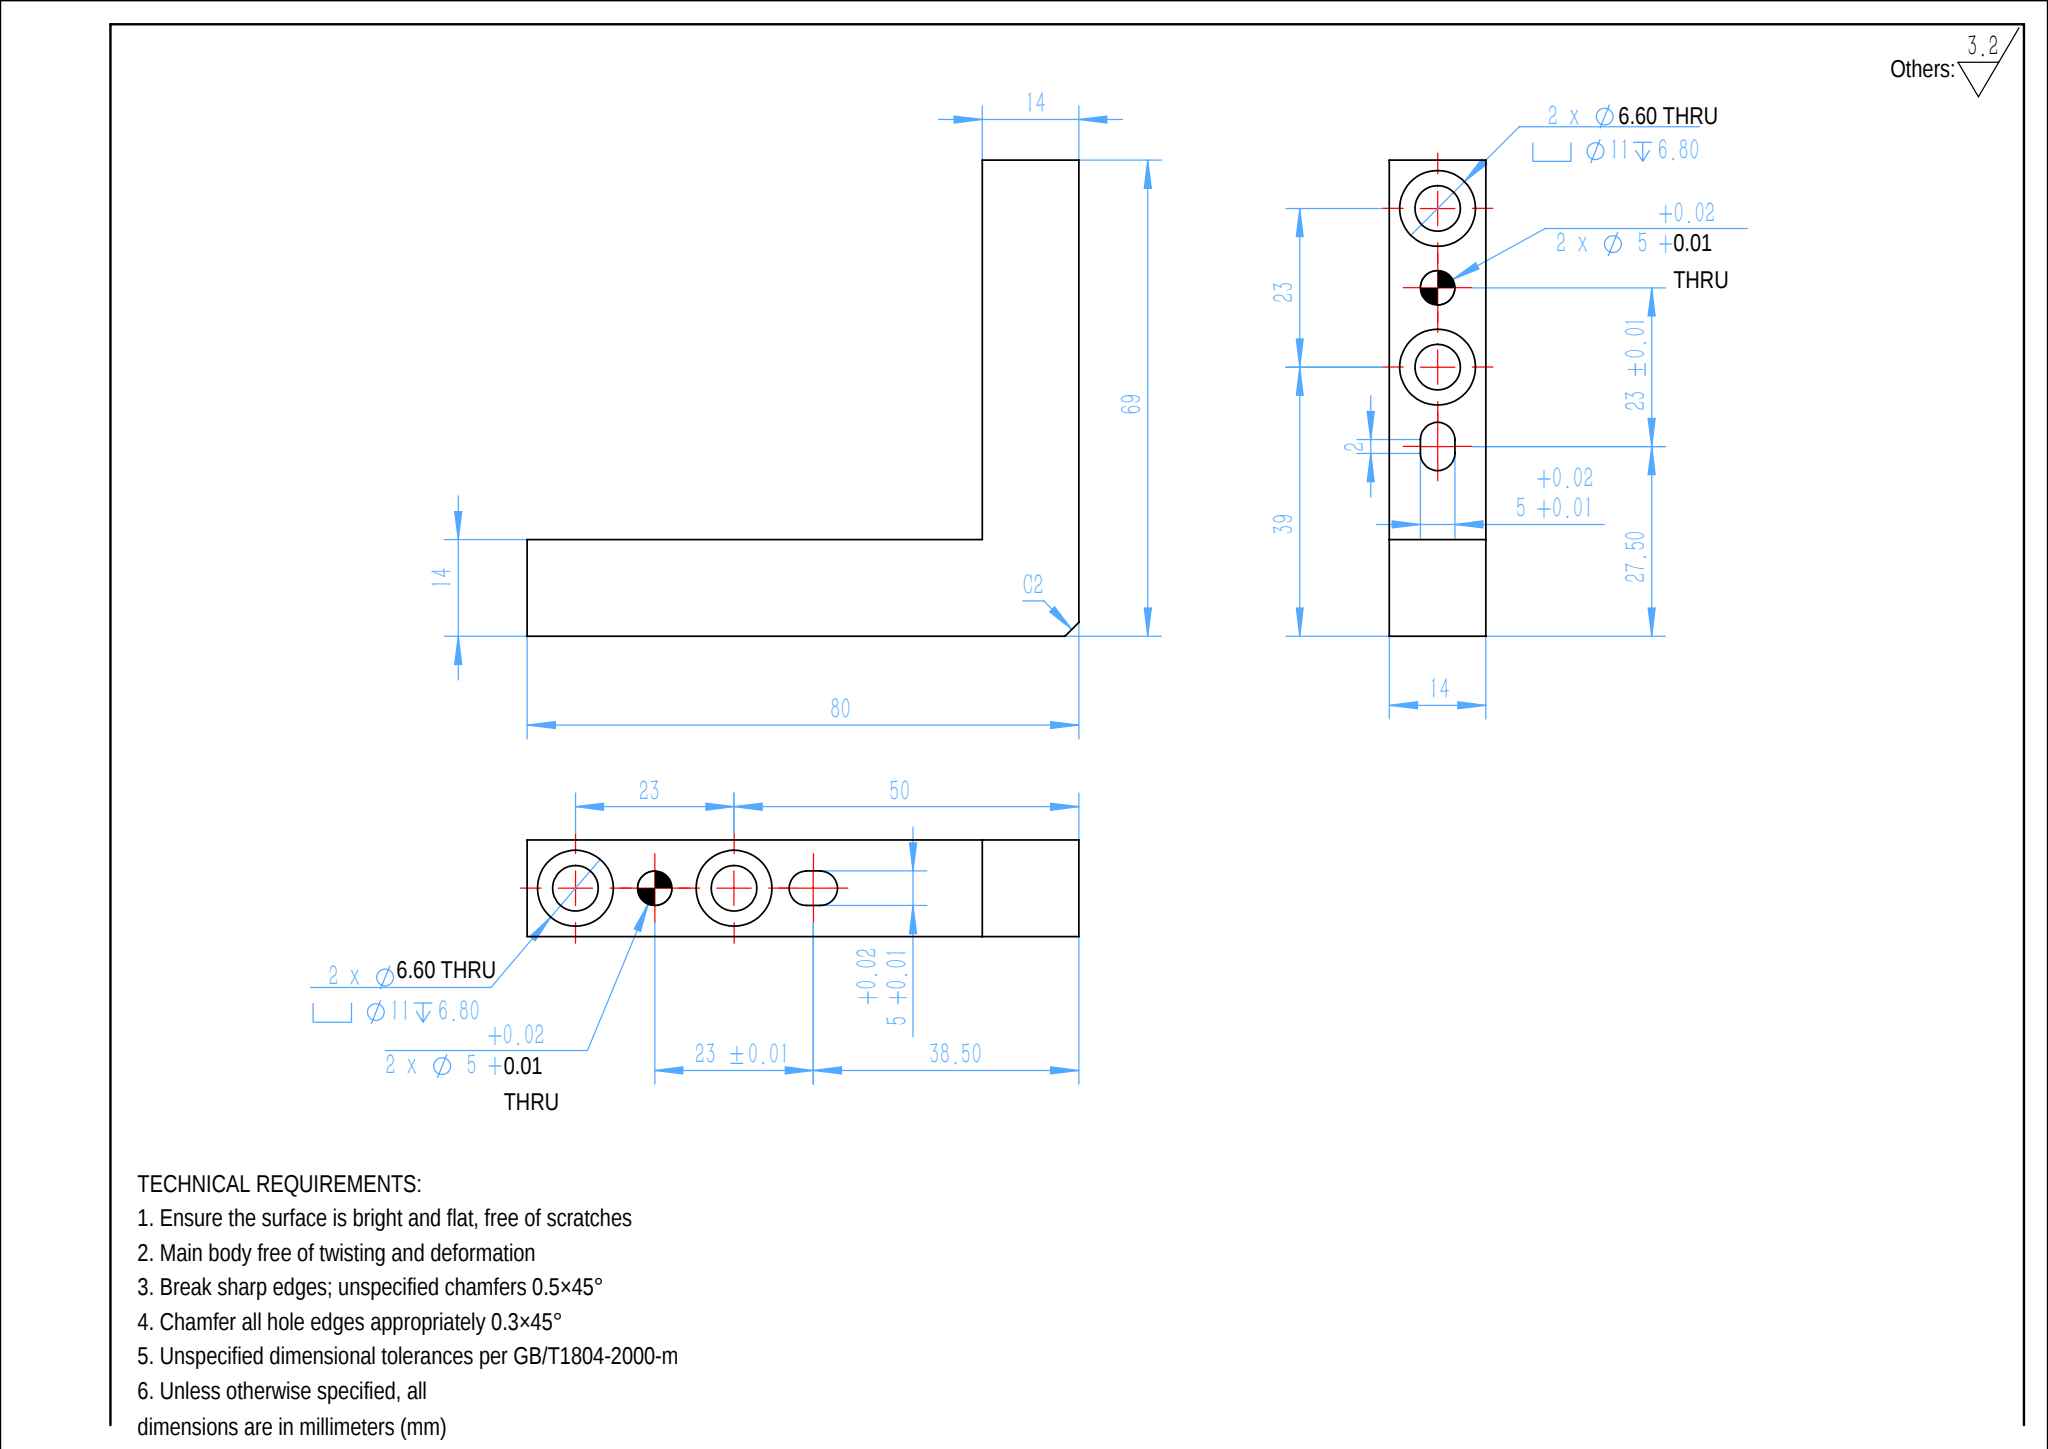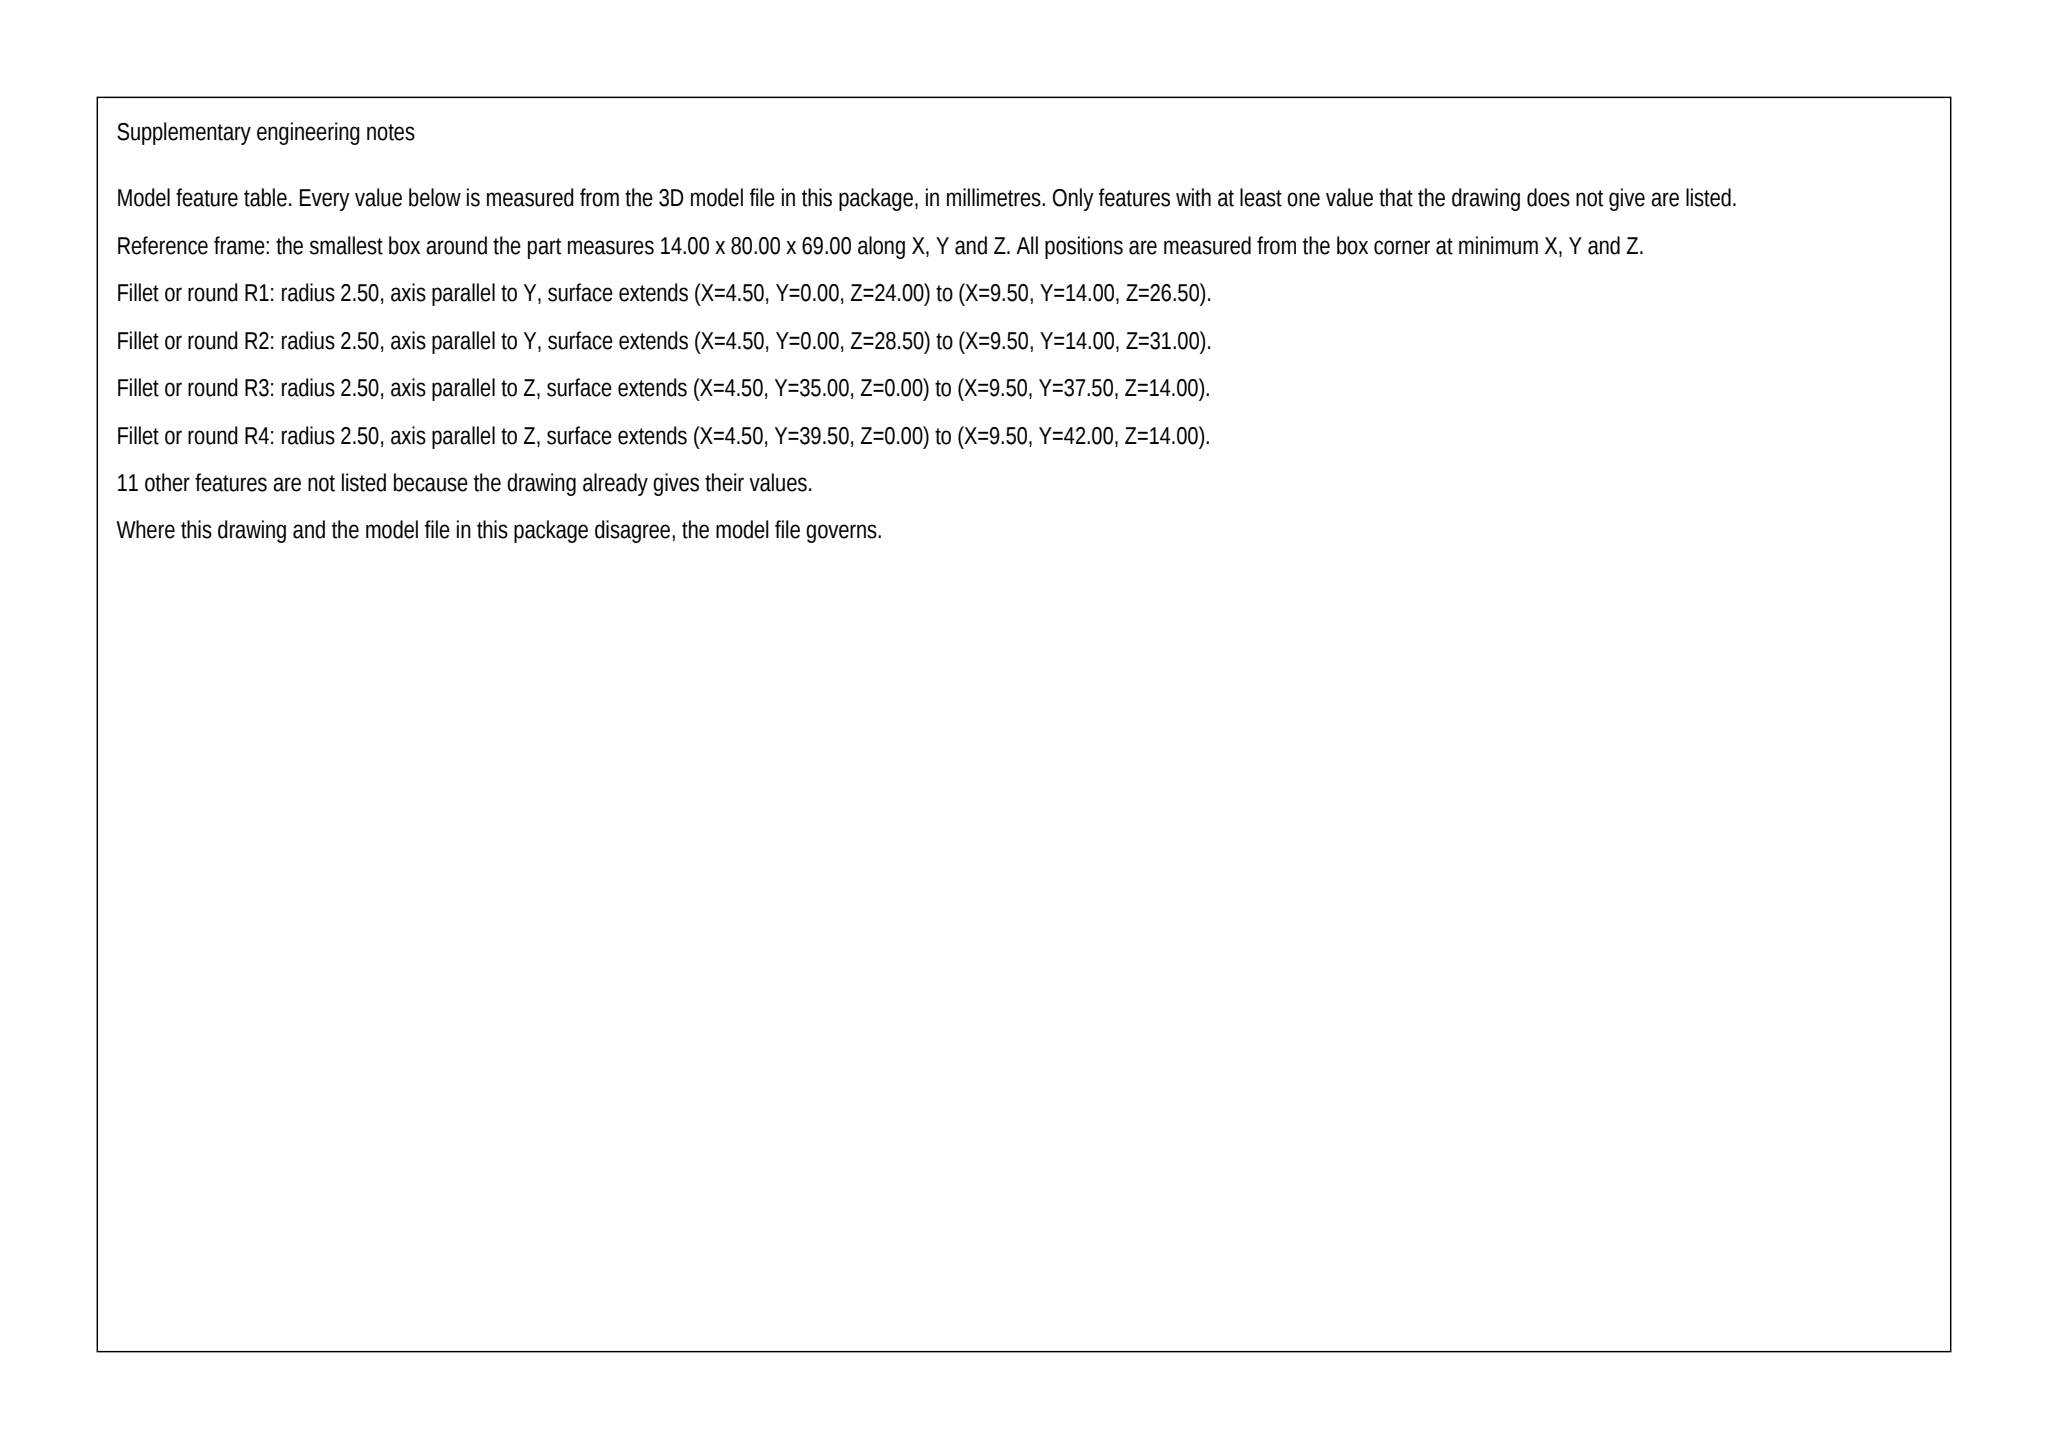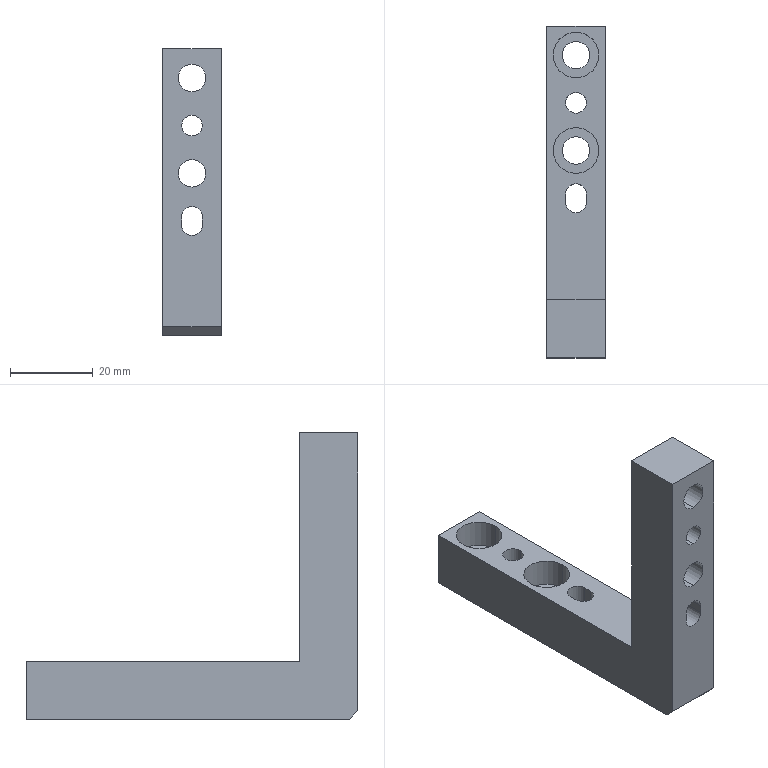Part | SolidWorks | mm | 1 solid | 42 faces | box 14 x 80 x 69 mm | volume 21482 mm3 | cylinder 25 | plane 17 | commonest cylinder face diameters 5 x9 11 x8 6.6 x8
build123d program:
from build123d import *

# Parameters (mm, degrees)
BOSS_EXTRUDE1_DEPTH                               = 7
HOLE_SIZE_ACCORDING_TO_TYPE_1_OF_HEXA_D           = 6.6
HOLE_SIZE_ACCORDING_TO_TYPE_1_OF_HEXA_CBORE_D     = 11
HOLE_SIZE_ACCORDING_TO_TYPE_1_OF_HEXA_CBORE_DEPTH = 6.8
HOLE_SIZE_ACCORDING_TO_TYPE_2_OF_HEXA_D           = 6.6
HOLE_SIZE_ACCORDING_TO_TYPE_2_OF_HEXA_CBORE_D     = 11
HOLE_SIZE_ACCORDING_TO_TYPE_2_OF_HEXA_CBORE_DEPTH = 6.8
F_5_0_5_DIAMETER_HOLE1_D                          = 5
F_5_0_5_DIAMETER_HOLE2_D                          = 5
CHAMFER1_SIZE                                     = 2
CUT_EXTRUDE1_DEPTH                                = 96.739
CUT_EXTRUDE2_DEPTH                                = 98.334


with BuildPart() as part:
    # Sketch1 → Boss-Extrude1 (new, symmetric)
    with BuildSketch(Plane(origin=(0, 0, 0), x_dir=(0, 0, -1), z_dir=(1, 0, 0))):
        Polygon((0, 0), (0, 80), (-14, 80), (-14, 25), (-14, 14), (-69, 14), (-69, 0), align=None)
    extrude(amount=BOSS_EXTRUDE1_DEPTH, both=True)

    # Hole Size _ according to_ Type 1 of Hexa (through all)
    with Locations(Plane.XY.offset(14)):
        with Locations((0, 73), (0, 50)):
            CounterBoreHole(HOLE_SIZE_ACCORDING_TO_TYPE_1_OF_HEXA_D / 2, HOLE_SIZE_ACCORDING_TO_TYPE_1_OF_HEXA_CBORE_D / 2, HOLE_SIZE_ACCORDING_TO_TYPE_1_OF_HEXA_CBORE_DEPTH)

    # Hole Size _ according to_ Type 2 of Hexa (through all)
    with Locations(Plane(origin=(0, 14, 0), x_dir=(-1, 0, 0), z_dir=(0, 1, 0))):
        with Locations((0, 39), (0, 62)):
            CounterBoreHole(HOLE_SIZE_ACCORDING_TO_TYPE_2_OF_HEXA_D / 2, HOLE_SIZE_ACCORDING_TO_TYPE_2_OF_HEXA_CBORE_D / 2, HOLE_SIZE_ACCORDING_TO_TYPE_2_OF_HEXA_CBORE_DEPTH)

    # 5.0 _5_ Diameter Hole1 (through all)
    with Locations(Plane(origin=(0, 0, 0), x_dir=(-1, 0, 0), z_dir=(0, 0, -1))):
        with Locations((0, 61.5), (0, 38.5)):
            Hole(F_5_0_5_DIAMETER_HOLE1_D / 2)

    # 5.0 _5_ Diameter Hole2 (through all)
    with Locations(Plane(origin=(0, 0, 0), x_dir=(-1, 0, 0), z_dir=(0, -1, 0))):
        with Locations((0, -50.5), (0, -27.5)):
            Hole(F_5_0_5_DIAMETER_HOLE2_D / 2)

    # Chamfer1
    chamfer1_edges = [part.edges().sort_by_distance(p)[0] for p in [
        (0, 0, 0),
    ]]
    chamfer(chamfer1_edges, length=CHAMFER1_SIZE)

    # Sketch10 → Cut-Extrude1 (cut, through all)
    with BuildSketch(Plane(origin=(0, 14, 0), x_dir=(1, 0, 0), z_dir=(0, 1, 0))):
        with BuildLine():
            Line((2.5, -26.5), (2.5, -28.5))
            ThreePointArc((2.5, -28.5), (0, -31), (-2.5, -28.5))
            Line((-2.5, -28.5), (-2.5, -26.5))
            ThreePointArc((-2.5, -26.5), (0, -24), (2.5, -26.5))
        make_face()
    extrude(amount=-CUT_EXTRUDE1_DEPTH, mode=Mode.SUBTRACT)

    # Sketch11 → Cut-Extrude2 (cut, through all)
    with BuildSketch(Plane.XY.offset(14)):
        with BuildLine():
            Line((-2.5, 37.5), (-2.5, 39.5))
            ThreePointArc((-2.5, 39.5), (0, 42), (2.5, 39.5))
            Line((2.5, 39.5), (2.5, 37.5))
            ThreePointArc((2.5, 37.5), (0, 35), (-2.5, 37.5))
        make_face()
    extrude(amount=-CUT_EXTRUDE2_DEPTH, mode=Mode.SUBTRACT)


solid = part.part